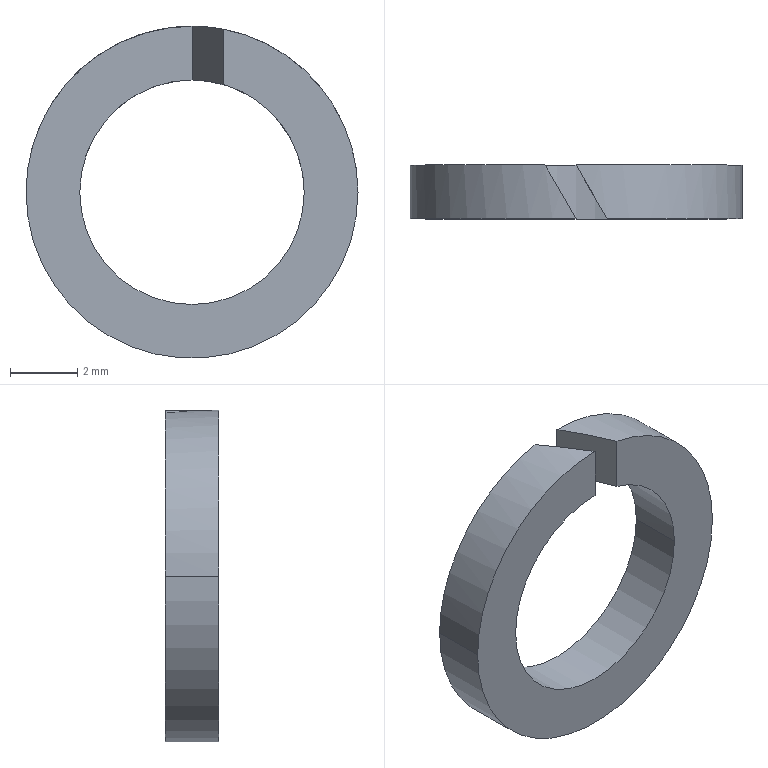Component | SolidWorks | spring lock washers--normal type gb-12 | 1 solid | 10 faces | volume 64 mm3 | cylinder 6 | plane 4 | commonest cylinder face diameters 6.68 x3 9.88 x3